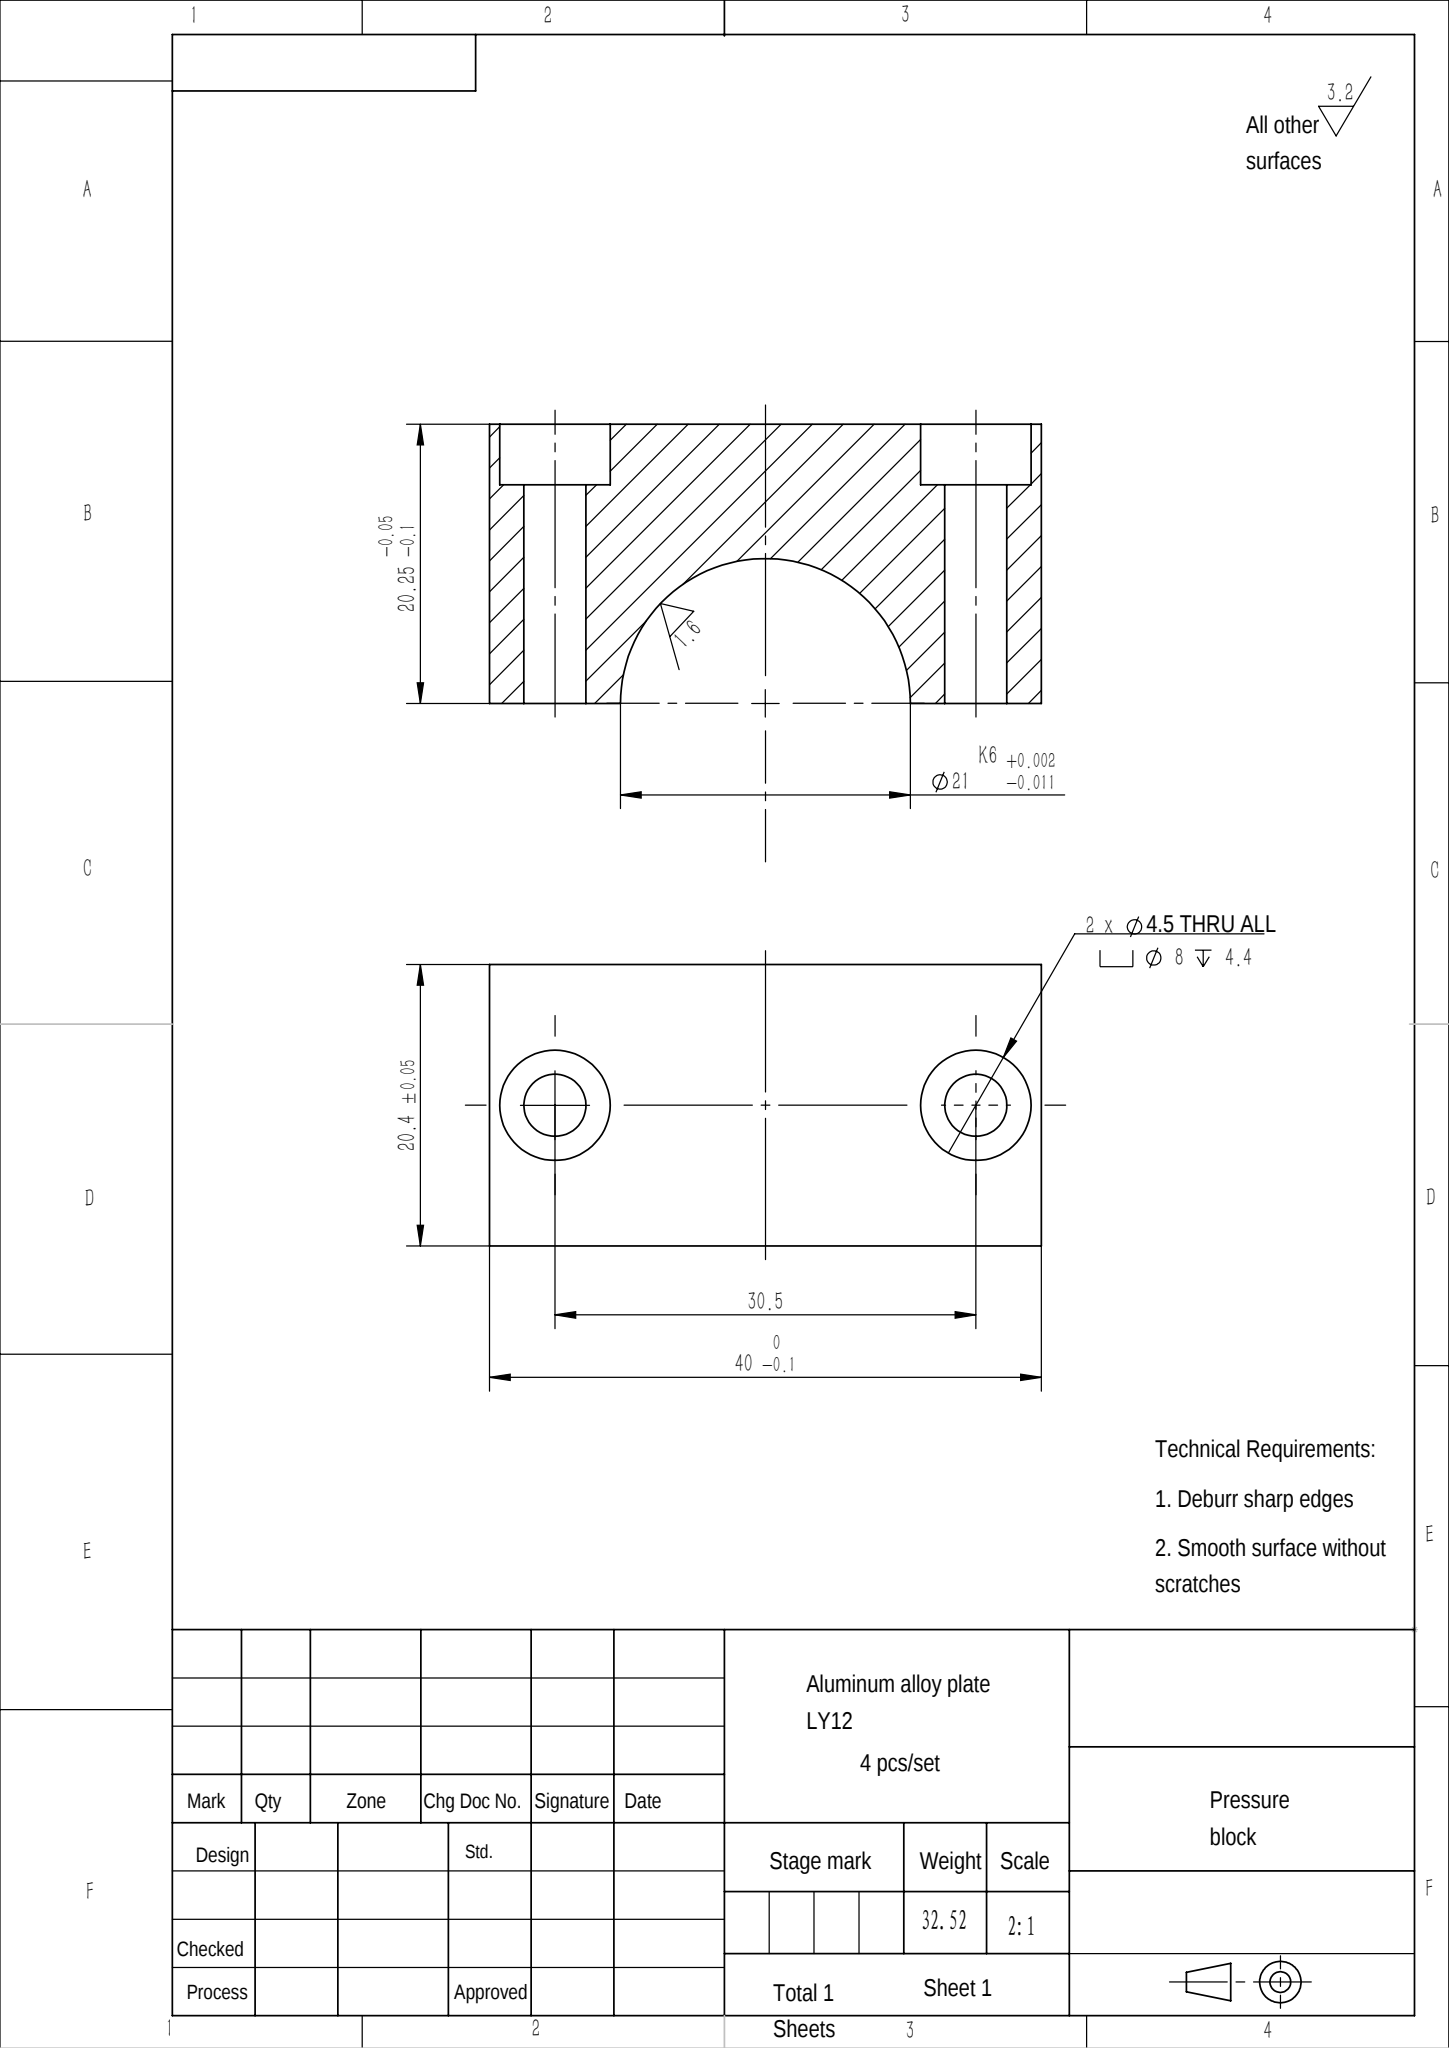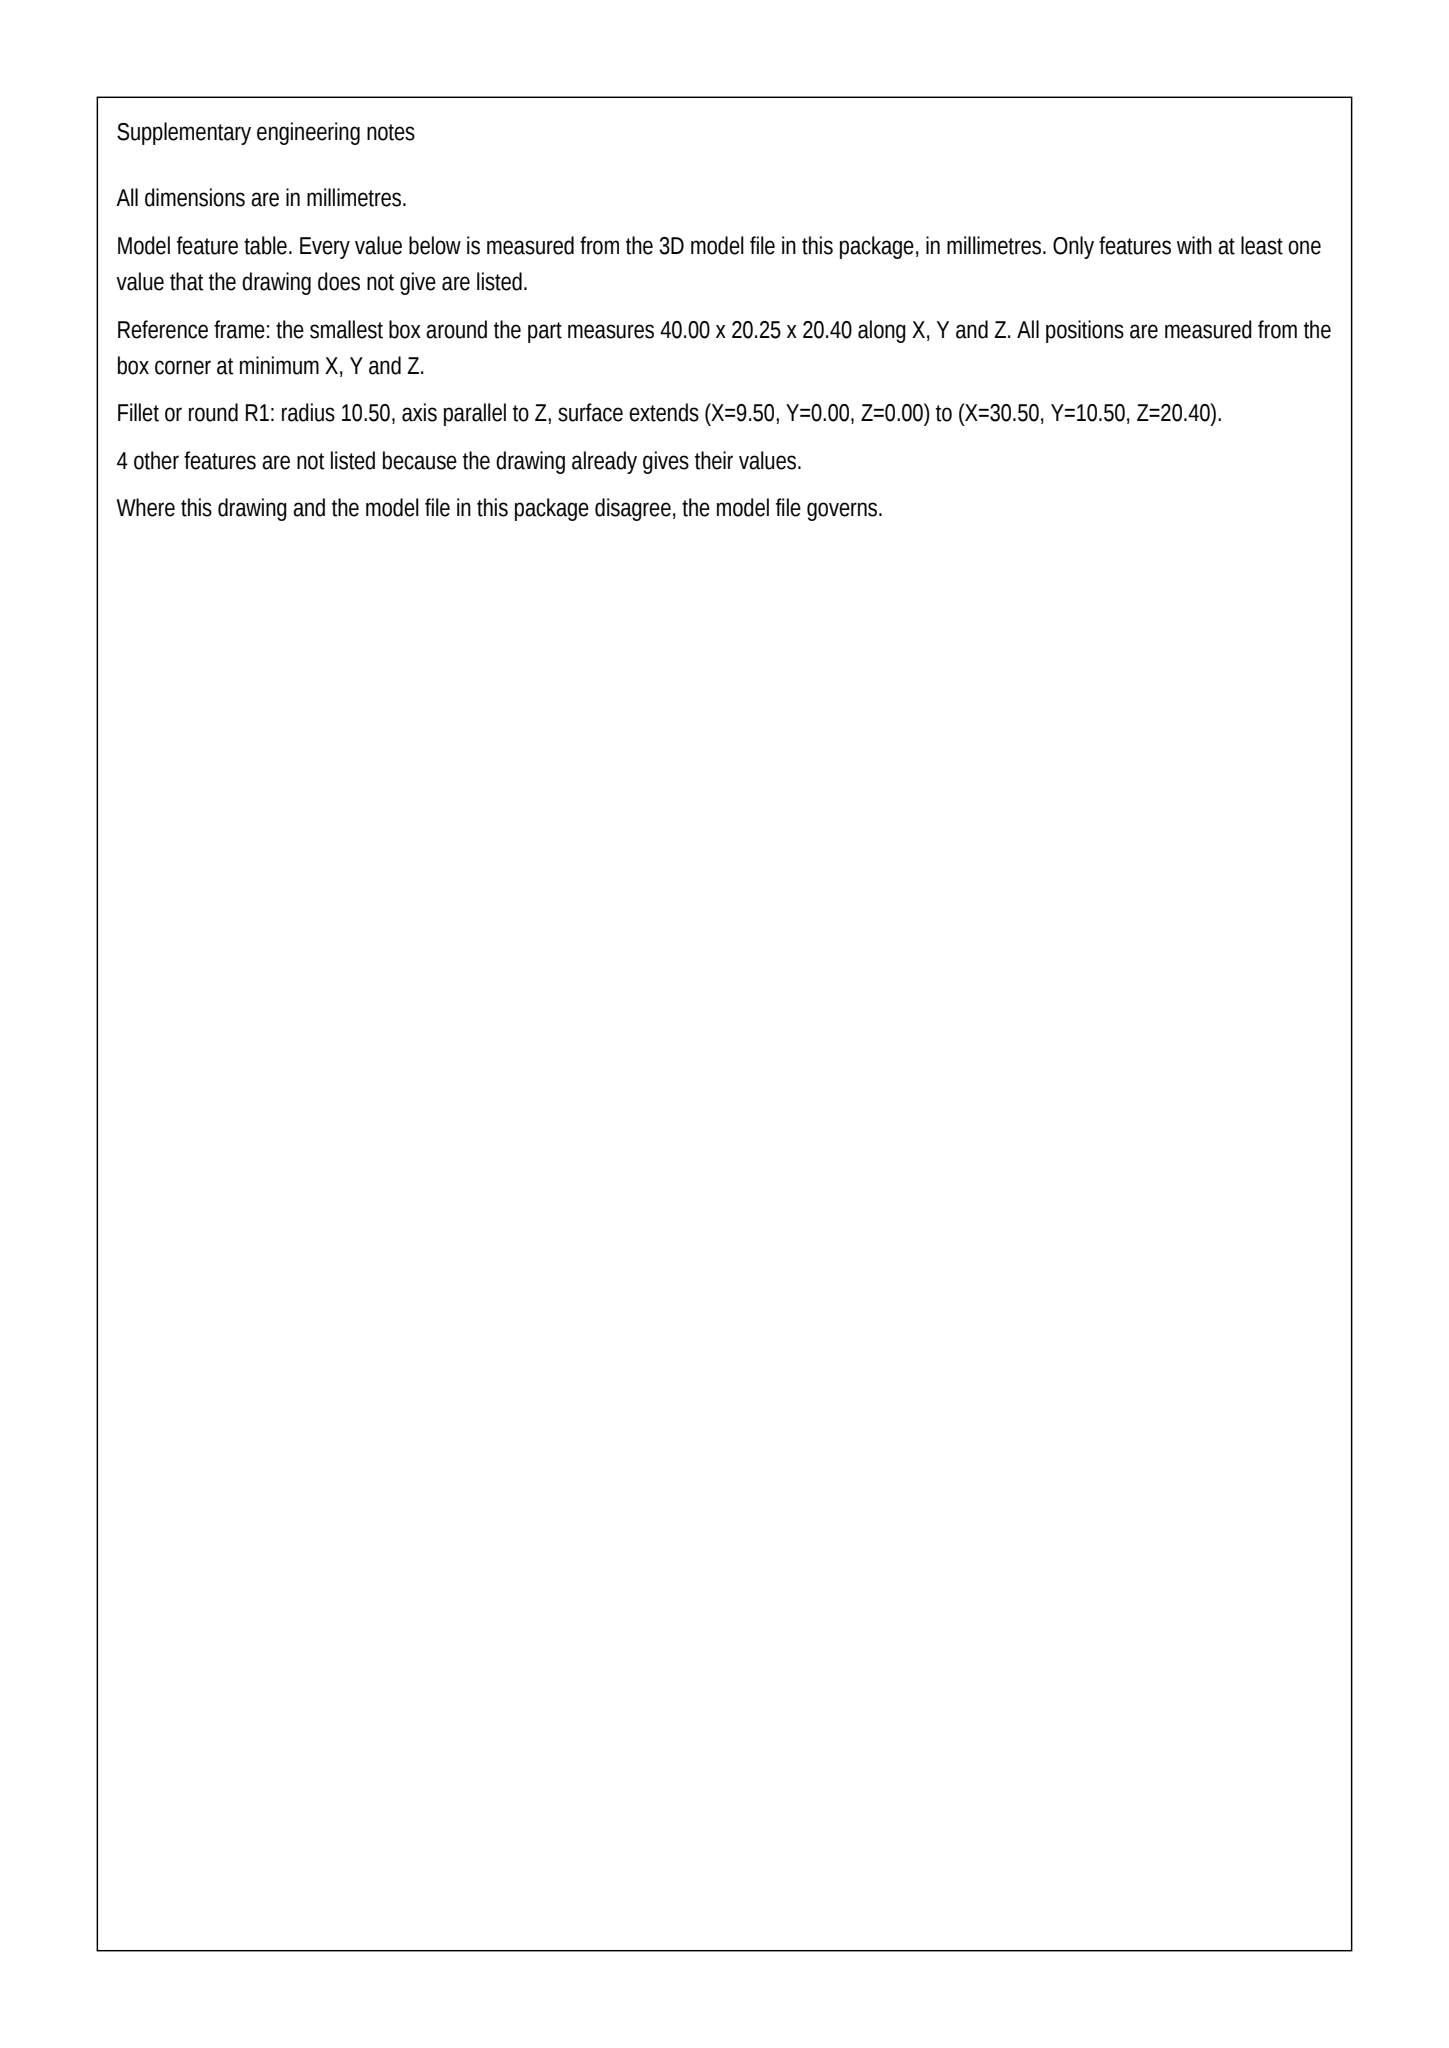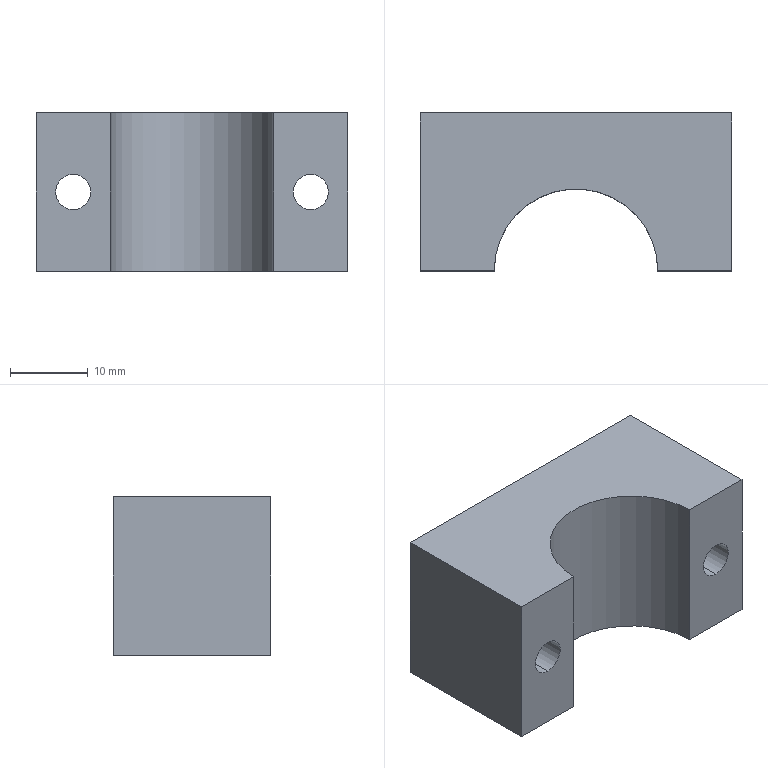Part | SolidWorks | mm | material Aluminum alloy plate LY12 | 1 solid | 18 faces | box 40 x 20.25 x 20.4 mm | volume 12045 mm3 | cylinder 9 | plane 9 | commonest cylinder face diameters 8 x4 4.5 x4 21 x1
build123d program:
from build123d import *

# Parameters (mm, degrees)
SKETCH1_W                                       = 40
SKETCH1_H                                       = 20.25
BOSS_EXTRUDE1_DEPTH                             = 10.2
SKETCH2_R                                       = 10.5
CUT_EXTRUDE1_DEPTH                              = 31.31
M4_HEX_SOCKET_HEAD_CAP_SCREW_CBORE1_D           = 4.5
M4_HEX_SOCKET_HEAD_CAP_SCREW_CBORE1_CBORE_D     = 8
M4_HEX_SOCKET_HEAD_CAP_SCREW_CBORE1_CBORE_DEPTH = 4.4


with BuildPart() as part:
    # Sketch1 → Boss-Extrude1 (new, symmetric)
    with BuildSketch(Plane.XY):
        Rectangle(SKETCH1_W, SKETCH1_H)
    extrude(amount=BOSS_EXTRUDE1_DEPTH, both=True)

    # Sketch2 → Cut-Extrude1 (cut, through all)
    with BuildSketch(Plane.XY.offset(10.2)):
        with Locations((0, -10.125)):
            Circle(SKETCH2_R)
    extrude(amount=-CUT_EXTRUDE1_DEPTH, mode=Mode.SUBTRACT)

    # M4 Hex Socket Head Cap Screw CBORE1 (through all)
    with Locations(Plane(origin=(0, 10.125, 0), x_dir=(1, 0, 0), z_dir=(0, 1, 0))):
        with Locations((-15.25, 0), (15.25, 0)):
            CounterBoreHole(M4_HEX_SOCKET_HEAD_CAP_SCREW_CBORE1_D / 2, M4_HEX_SOCKET_HEAD_CAP_SCREW_CBORE1_CBORE_D / 2, M4_HEX_SOCKET_HEAD_CAP_SCREW_CBORE1_CBORE_DEPTH)


solid = part.part
STEP:
#1=CARTESIAN_POINT('',(-15.25,5.725,-4.));
#2=VERTEX_POINT('',#1);
#3=CARTESIAN_POINT('',(-15.25,5.725,4.));
#4=VERTEX_POINT('',#3);
#5=CARTESIAN_POINT('',(-15.25,5.725,0.));
#6=DIRECTION('',(0.,1.,0.));
#7=DIRECTION('',(0.,0.,1.));
#8=AXIS2_PLACEMENT_3D('',#5,#6,#7);
#9=CIRCLE('',#8,4.);
#10=EDGE_CURVE('',#2,#4,#9,.T.);
#11=ORIENTED_EDGE('',*,*,#10,.F.);
#12=CARTESIAN_POINT('',(-15.25,10.125,-4.));
#13=VERTEX_POINT('',#12);
#14=CARTESIAN_POINT('',(-15.25,10.125,-4.));
#15=DIRECTION('',(0.,1.,0.));
#16=VECTOR('',#15,1000.);
#17=LINE('',#14,#16);
#18=EDGE_CURVE('',#2,#13,#17,.T.);
#19=ORIENTED_EDGE('',*,*,#18,.T.);
#20=CARTESIAN_POINT('',(-15.25,10.125,4.));
#21=VERTEX_POINT('',#20);
#22=CARTESIAN_POINT('',(-15.25,10.125,0.));
#23=DIRECTION('',(0.,1.,0.));
#24=DIRECTION('',(0.,0.,1.));
#25=AXIS2_PLACEMENT_3D('',#22,#23,#24);
#26=CIRCLE('',#25,4.);
#27=EDGE_CURVE('',#13,#21,#26,.T.);
#28=ORIENTED_EDGE('',*,*,#27,.T.);
#29=CARTESIAN_POINT('',(-15.25,10.125,4.));
#30=DIRECTION('',(0.,1.,0.));
#31=VECTOR('',#30,1000.);
#32=LINE('',#29,#31);
#33=EDGE_CURVE('',#4,#21,#32,.T.);
#34=ORIENTED_EDGE('',*,*,#33,.F.);
#35=EDGE_LOOP('',(#11,#19,#28,#34));
#36=FACE_OUTER_BOUND('',#35,.T.);
#37=CARTESIAN_POINT('',(-15.25,10.125,0.));
#38=DIRECTION('',(0.,1.,0.));
#39=DIRECTION('',(0.,0.,1.));
#40=AXIS2_PLACEMENT_3D('',#37,#38,#39);
#41=CYLINDRICAL_SURFACE('',#40,4.);
#42=ADVANCED_FACE('',(#36),#41,.F.);
#43=CARTESIAN_POINT('',(-15.25,-10.125,-2.25));
#44=VERTEX_POINT('',#43);
#45=CARTESIAN_POINT('',(-15.25,-10.125,2.25));
#46=VERTEX_POINT('',#45);
#47=CARTESIAN_POINT('',(-15.25,-10.125,0.));
#48=DIRECTION('',(0.,1.,0.));
#49=DIRECTION('',(0.,0.,1.));
#50=AXIS2_PLACEMENT_3D('',#47,#48,#49);
#51=CIRCLE('',#50,2.25);
#52=EDGE_CURVE('',#44,#46,#51,.T.);
#53=ORIENTED_EDGE('',*,*,#52,.F.);
#54=CARTESIAN_POINT('',(-15.25,5.725,-2.25));
#55=VERTEX_POINT('',#54);
#56=CARTESIAN_POINT('',(-15.25,10.125,-2.25));
#57=DIRECTION('',(0.,1.,0.));
#58=VECTOR('',#57,1000.);
#59=LINE('',#56,#58);
#60=EDGE_CURVE('',#44,#55,#59,.T.);
#61=ORIENTED_EDGE('',*,*,#60,.T.);
#62=CARTESIAN_POINT('',(-15.25,5.725,2.25));
#63=VERTEX_POINT('',#62);
#64=CARTESIAN_POINT('',(-15.25,5.725,0.));
#65=DIRECTION('',(0.,1.,0.));
#66=DIRECTION('',(0.,0.,1.));
#67=AXIS2_PLACEMENT_3D('',#64,#65,#66);
#68=CIRCLE('',#67,2.25);
#69=EDGE_CURVE('',#55,#63,#68,.T.);
#70=ORIENTED_EDGE('',*,*,#69,.T.);
#71=CARTESIAN_POINT('',(-15.25,10.125,2.25));
#72=DIRECTION('',(0.,1.,0.));
#73=VECTOR('',#72,1000.);
#74=LINE('',#71,#73);
#75=EDGE_CURVE('',#46,#63,#74,.T.);
#76=ORIENTED_EDGE('',*,*,#75,.F.);
#77=EDGE_LOOP('',(#53,#61,#70,#76));
#78=FACE_OUTER_BOUND('',#77,.T.);
#79=CARTESIAN_POINT('',(-15.25,10.125,0.));
#80=DIRECTION('',(0.,1.,0.));
#81=DIRECTION('',(0.,0.,1.));
#82=AXIS2_PLACEMENT_3D('',#79,#80,#81);
#83=CYLINDRICAL_SURFACE('',#82,2.25);
#84=ADVANCED_FACE('',(#78),#83,.F.);
#85=CARTESIAN_POINT('',(15.25,5.725,-4.));
#86=VERTEX_POINT('',#85);
#87=CARTESIAN_POINT('',(15.25,5.725,4.));
#88=VERTEX_POINT('',#87);
#89=CARTESIAN_POINT('',(15.25,5.725,0.));
#90=DIRECTION('',(0.,1.,0.));
#91=DIRECTION('',(0.,0.,1.));
#92=AXIS2_PLACEMENT_3D('',#89,#90,#91);
#93=CIRCLE('',#92,4.);
#94=EDGE_CURVE('',#86,#88,#93,.T.);
#95=ORIENTED_EDGE('',*,*,#94,.F.);
#96=CARTESIAN_POINT('',(15.25,10.125,-4.));
#97=VERTEX_POINT('',#96);
#98=CARTESIAN_POINT('',(15.25,10.125,-4.));
#99=DIRECTION('',(0.,1.,0.));
#100=VECTOR('',#99,1000.);
#101=LINE('',#98,#100);
#102=EDGE_CURVE('',#86,#97,#101,.T.);
#103=ORIENTED_EDGE('',*,*,#102,.T.);
#104=CARTESIAN_POINT('',(15.25,10.125,4.));
#105=VERTEX_POINT('',#104);
#106=CARTESIAN_POINT('',(15.25,10.125,0.));
#107=DIRECTION('',(0.,1.,0.));
#108=DIRECTION('',(0.,0.,1.));
#109=AXIS2_PLACEMENT_3D('',#106,#107,#108);
#110=CIRCLE('',#109,4.);
#111=EDGE_CURVE('',#97,#105,#110,.T.);
#112=ORIENTED_EDGE('',*,*,#111,.T.);
#113=CARTESIAN_POINT('',(15.25,10.125,4.));
#114=DIRECTION('',(0.,1.,0.));
#115=VECTOR('',#114,1000.);
#116=LINE('',#113,#115);
#117=EDGE_CURVE('',#88,#105,#116,.T.);
#118=ORIENTED_EDGE('',*,*,#117,.F.);
#119=EDGE_LOOP('',(#95,#103,#112,#118));
#120=FACE_OUTER_BOUND('',#119,.T.);
#121=CARTESIAN_POINT('',(15.25,10.125,0.));
#122=DIRECTION('',(0.,1.,0.));
#123=DIRECTION('',(0.,0.,1.));
#124=AXIS2_PLACEMENT_3D('',#121,#122,#123);
#125=CYLINDRICAL_SURFACE('',#124,4.);
#126=ADVANCED_FACE('',(#120),#125,.F.);
#127=CARTESIAN_POINT('',(15.25,-10.125,-2.25));
#128=VERTEX_POINT('',#127);
#129=CARTESIAN_POINT('',(15.25,-10.125,2.25));
#130=VERTEX_POINT('',#129);
#131=CARTESIAN_POINT('',(15.25,-10.125,0.));
#132=DIRECTION('',(0.,1.,0.));
#133=DIRECTION('',(0.,0.,1.));
#134=AXIS2_PLACEMENT_3D('',#131,#132,#133);
#135=CIRCLE('',#134,2.25);
#136=EDGE_CURVE('',#128,#130,#135,.T.);
#137=ORIENTED_EDGE('',*,*,#136,.F.);
#138=CARTESIAN_POINT('',(15.25,5.725,-2.25));
#139=VERTEX_POINT('',#138);
#140=CARTESIAN_POINT('',(15.25,10.125,-2.25));
#141=DIRECTION('',(0.,1.,0.));
#142=VECTOR('',#141,1000.);
#143=LINE('',#140,#142);
#144=EDGE_CURVE('',#128,#139,#143,.T.);
#145=ORIENTED_EDGE('',*,*,#144,.T.);
#146=CARTESIAN_POINT('',(15.25,5.725,2.25));
#147=VERTEX_POINT('',#146);
#148=CARTESIAN_POINT('',(15.25,5.725,0.));
#149=DIRECTION('',(0.,1.,0.));
#150=DIRECTION('',(0.,0.,1.));
#151=AXIS2_PLACEMENT_3D('',#148,#149,#150);
#152=CIRCLE('',#151,2.25);
#153=EDGE_CURVE('',#139,#147,#152,.T.);
#154=ORIENTED_EDGE('',*,*,#153,.T.);
#155=CARTESIAN_POINT('',(15.25,10.125,2.25));
#156=DIRECTION('',(0.,1.,0.));
#157=VECTOR('',#156,1000.);
#158=LINE('',#155,#157);
#159=EDGE_CURVE('',#130,#147,#158,.T.);
#160=ORIENTED_EDGE('',*,*,#159,.F.);
#161=EDGE_LOOP('',(#137,#145,#154,#160));
#162=FACE_OUTER_BOUND('',#161,.T.);
#163=CARTESIAN_POINT('',(15.25,10.125,0.));
#164=DIRECTION('',(0.,1.,0.));
#165=DIRECTION('',(0.,0.,1.));
#166=AXIS2_PLACEMENT_3D('',#163,#164,#165);
#167=CYLINDRICAL_SURFACE('',#166,2.25);
#168=ADVANCED_FACE('',(#162),#167,.F.);
#169=CARTESIAN_POINT('',(-15.25,-10.125,0.));
#170=DIRECTION('',(0.,1.,0.));
#171=DIRECTION('',(0.,0.,1.));
#172=AXIS2_PLACEMENT_3D('',#169,#170,#171);
#173=CIRCLE('',#172,2.25);
#174=EDGE_CURVE('',#46,#44,#173,.T.);
#175=ORIENTED_EDGE('',*,*,#174,.T.);
#176=ORIENTED_EDGE('',*,*,#52,.T.);
#177=EDGE_LOOP('',(#175,#176));
#178=FACE_BOUND('',#177,.T.);
#179=CARTESIAN_POINT('',(-20.,-10.125,-10.2));
#180=VERTEX_POINT('',#179);
#181=CARTESIAN_POINT('',(-10.5,-10.125,-10.2));
#182=VERTEX_POINT('',#181);
#183=CARTESIAN_POINT('',(-20.,-10.125,-10.2));
#184=DIRECTION('',(1.,0.,0.));
#185=VECTOR('',#184,1000.);
#186=LINE('',#183,#185);
#187=EDGE_CURVE('',#180,#182,#186,.T.);
#188=ORIENTED_EDGE('',*,*,#187,.T.);
#189=CARTESIAN_POINT('',(-10.5,-10.125,10.2));
#190=VERTEX_POINT('',#189);
#191=CARTESIAN_POINT('',(-10.5,-10.125,-10.2));
#192=DIRECTION('',(0.,0.,1.));
#193=VECTOR('',#192,1000.);
#194=LINE('',#191,#193);
#195=EDGE_CURVE('',#182,#190,#194,.T.);
#196=ORIENTED_EDGE('',*,*,#195,.T.);
#197=CARTESIAN_POINT('',(-20.,-10.125,10.2));
#198=VERTEX_POINT('',#197);
#199=CARTESIAN_POINT('',(-20.,-10.125,10.2));
#200=DIRECTION('',(1.,0.,0.));
#201=VECTOR('',#200,1000.);
#202=LINE('',#199,#201);
#203=EDGE_CURVE('',#198,#190,#202,.T.);
#204=ORIENTED_EDGE('',*,*,#203,.F.);
#205=CARTESIAN_POINT('',(-20.,-10.125,10.2));
#206=DIRECTION('',(0.,0.,-1.));
#207=VECTOR('',#206,1000.);
#208=LINE('',#205,#207);
#209=EDGE_CURVE('',#198,#180,#208,.T.);
#210=ORIENTED_EDGE('',*,*,#209,.T.);
#211=EDGE_LOOP('',(#188,#196,#204,#210));
#212=FACE_OUTER_BOUND('',#211,.T.);
#213=CARTESIAN_POINT('',(-20.,-10.125,10.2));
#214=DIRECTION('',(0.,1.,0.));
#215=DIRECTION('',(0.,0.,1.));
#216=AXIS2_PLACEMENT_3D('',#213,#214,#215);
#217=PLANE('',#216);
#218=ADVANCED_FACE('',(#178,#212),#217,.F.);
#219=CARTESIAN_POINT('',(20.,-10.125,-10.2));
#220=VERTEX_POINT('',#219);
#221=CARTESIAN_POINT('',(20.,10.125,-10.2));
#222=VERTEX_POINT('',#221);
#223=CARTESIAN_POINT('',(20.,10.125,-10.2));
#224=DIRECTION('',(0.,1.,0.));
#225=VECTOR('',#224,1000.);
#226=LINE('',#223,#225);
#227=EDGE_CURVE('',#220,#222,#226,.T.);
#228=ORIENTED_EDGE('',*,*,#227,.T.);
#229=CARTESIAN_POINT('',(20.,10.125,10.2));
#230=VERTEX_POINT('',#229);
#231=CARTESIAN_POINT('',(20.,10.125,10.2));
#232=DIRECTION('',(0.,0.,-1.));
#233=VECTOR('',#232,1000.);
#234=LINE('',#231,#233);
#235=EDGE_CURVE('',#230,#222,#234,.T.);
#236=ORIENTED_EDGE('',*,*,#235,.F.);
#237=CARTESIAN_POINT('',(20.,-10.125,10.2));
#238=VERTEX_POINT('',#237);
#239=CARTESIAN_POINT('',(20.,10.125,10.2));
#240=DIRECTION('',(0.,1.,0.));
#241=VECTOR('',#240,1000.);
#242=LINE('',#239,#241);
#243=EDGE_CURVE('',#238,#230,#242,.T.);
#244=ORIENTED_EDGE('',*,*,#243,.F.);
#245=CARTESIAN_POINT('',(20.,-10.125,10.2));
#246=DIRECTION('',(0.,0.,-1.));
#247=VECTOR('',#246,1000.);
#248=LINE('',#245,#247);
#249=EDGE_CURVE('',#238,#220,#248,.T.);
#250=ORIENTED_EDGE('',*,*,#249,.T.);
#251=EDGE_LOOP('',(#228,#236,#244,#250));
#252=FACE_OUTER_BOUND('',#251,.T.);
#253=CARTESIAN_POINT('',(20.,10.125,10.2));
#254=DIRECTION('',(-1.,0.,0.));
#255=DIRECTION('',(0.,0.,1.));
#256=AXIS2_PLACEMENT_3D('',#253,#254,#255);
#257=PLANE('',#256);
#258=ADVANCED_FACE('',(#252),#257,.F.);
#259=CARTESIAN_POINT('',(-15.25,10.125,0.));
#260=DIRECTION('',(0.,1.,0.));
#261=DIRECTION('',(0.,0.,1.));
#262=AXIS2_PLACEMENT_3D('',#259,#260,#261);
#263=CIRCLE('',#262,4.);
#264=EDGE_CURVE('',#21,#13,#263,.T.);
#265=ORIENTED_EDGE('',*,*,#264,.F.);
#266=ORIENTED_EDGE('',*,*,#27,.F.);
#267=EDGE_LOOP('',(#265,#266));
#268=FACE_BOUND('',#267,.T.);
#269=CARTESIAN_POINT('',(15.25,10.125,0.));
#270=DIRECTION('',(0.,1.,0.));
#271=DIRECTION('',(0.,0.,1.));
#272=AXIS2_PLACEMENT_3D('',#269,#270,#271);
#273=CIRCLE('',#272,4.);
#274=EDGE_CURVE('',#105,#97,#273,.T.);
#275=ORIENTED_EDGE('',*,*,#274,.F.);
#276=ORIENTED_EDGE('',*,*,#111,.F.);
#277=EDGE_LOOP('',(#275,#276));
#278=FACE_BOUND('',#277,.T.);
#279=CARTESIAN_POINT('',(-20.,10.125,-10.2));
#280=VERTEX_POINT('',#279);
#281=CARTESIAN_POINT('',(-20.,10.125,-10.2));
#282=DIRECTION('',(-1.,0.,0.));
#283=VECTOR('',#282,1000.);
#284=LINE('',#281,#283);
#285=EDGE_CURVE('',#222,#280,#284,.T.);
#286=ORIENTED_EDGE('',*,*,#285,.T.);
#287=CARTESIAN_POINT('',(-20.,10.125,10.2));
#288=VERTEX_POINT('',#287);
#289=CARTESIAN_POINT('',(-20.,10.125,10.2));
#290=DIRECTION('',(0.,0.,-1.));
#291=VECTOR('',#290,1000.);
#292=LINE('',#289,#291);
#293=EDGE_CURVE('',#288,#280,#292,.T.);
#294=ORIENTED_EDGE('',*,*,#293,.F.);
#295=CARTESIAN_POINT('',(-20.,10.125,10.2));
#296=DIRECTION('',(-1.,0.,0.));
#297=VECTOR('',#296,1000.);
#298=LINE('',#295,#297);
#299=EDGE_CURVE('',#230,#288,#298,.T.);
#300=ORIENTED_EDGE('',*,*,#299,.F.);
#301=ORIENTED_EDGE('',*,*,#235,.T.);
#302=EDGE_LOOP('',(#286,#294,#300,#301));
#303=FACE_OUTER_BOUND('',#302,.T.);
#304=CARTESIAN_POINT('',(-20.,10.125,10.2));
#305=DIRECTION('',(0.,-1.,0.));
#306=DIRECTION('',(0.,0.,-1.));
#307=AXIS2_PLACEMENT_3D('',#304,#305,#306);
#308=PLANE('',#307);
#309=ADVANCED_FACE('',(#268,#278,#303),#308,.F.);
#310=CARTESIAN_POINT('',(-20.,10.125,-10.2));
#311=DIRECTION('',(0.,-1.,0.));
#312=VECTOR('',#311,1000.);
#313=LINE('',#310,#312);
#314=EDGE_CURVE('',#280,#180,#313,.T.);
#315=ORIENTED_EDGE('',*,*,#314,.T.);
#316=ORIENTED_EDGE('',*,*,#209,.F.);
#317=CARTESIAN_POINT('',(-20.,10.125,10.2));
#318=DIRECTION('',(0.,-1.,0.));
#319=VECTOR('',#318,1000.);
#320=LINE('',#317,#319);
#321=EDGE_CURVE('',#288,#198,#320,.T.);
#322=ORIENTED_EDGE('',*,*,#321,.F.);
#323=ORIENTED_EDGE('',*,*,#293,.T.);
#324=EDGE_LOOP('',(#315,#316,#322,#323));
#325=FACE_OUTER_BOUND('',#324,.T.);
#326=CARTESIAN_POINT('',(-20.,10.125,10.2));
#327=DIRECTION('',(1.,0.,0.));
#328=DIRECTION('',(0.,0.,-1.));
#329=AXIS2_PLACEMENT_3D('',#326,#327,#328);
#330=PLANE('',#329);
#331=ADVANCED_FACE('',(#325),#330,.F.);
#332=CARTESIAN_POINT('',(15.25,-10.125,0.));
#333=DIRECTION('',(0.,1.,0.));
#334=DIRECTION('',(0.,0.,1.));
#335=AXIS2_PLACEMENT_3D('',#332,#333,#334);
#336=CIRCLE('',#335,2.25);
#337=EDGE_CURVE('',#130,#128,#336,.T.);
#338=ORIENTED_EDGE('',*,*,#337,.T.);
#339=ORIENTED_EDGE('',*,*,#136,.T.);
#340=EDGE_LOOP('',(#338,#339));
#341=FACE_BOUND('',#340,.T.);
#342=CARTESIAN_POINT('',(10.5,-10.125,10.2));
#343=VERTEX_POINT('',#342);
#344=CARTESIAN_POINT('',(-20.,-10.125,10.2));
#345=DIRECTION('',(1.,0.,0.));
#346=VECTOR('',#345,1000.);
#347=LINE('',#344,#346);
#348=EDGE_CURVE('',#343,#238,#347,.T.);
#349=ORIENTED_EDGE('',*,*,#348,.F.);
#350=CARTESIAN_POINT('',(10.5,-10.125,-10.2));
#351=VERTEX_POINT('',#350);
#352=CARTESIAN_POINT('',(10.5,-10.125,-10.2));
#353=DIRECTION('',(0.,0.,-1.));
#354=VECTOR('',#353,1000.);
#355=LINE('',#352,#354);
#356=EDGE_CURVE('',#343,#351,#355,.T.);
#357=ORIENTED_EDGE('',*,*,#356,.T.);
#358=CARTESIAN_POINT('',(-20.,-10.125,-10.2));
#359=DIRECTION('',(1.,0.,0.));
#360=VECTOR('',#359,1000.);
#361=LINE('',#358,#360);
#362=EDGE_CURVE('',#351,#220,#361,.T.);
#363=ORIENTED_EDGE('',*,*,#362,.T.);
#364=ORIENTED_EDGE('',*,*,#249,.F.);
#365=EDGE_LOOP('',(#349,#357,#363,#364));
#366=FACE_OUTER_BOUND('',#365,.T.);
#367=CARTESIAN_POINT('',(-20.,-10.125,10.2));
#368=DIRECTION('',(0.,1.,0.));
#369=DIRECTION('',(0.,0.,1.));
#370=AXIS2_PLACEMENT_3D('',#367,#368,#369);
#371=PLANE('',#370);
#372=ADVANCED_FACE('',(#341,#366),#371,.F.);
#373=CARTESIAN_POINT('',(0.,-10.125,10.2));
#374=DIRECTION('',(0.,0.,1.));
#375=DIRECTION('',(1.,0.,0.));
#376=AXIS2_PLACEMENT_3D('',#373,#374,#375);
#377=CIRCLE('',#376,10.5);
#378=EDGE_CURVE('',#343,#190,#377,.T.);
#379=ORIENTED_EDGE('',*,*,#378,.F.);
#380=ORIENTED_EDGE('',*,*,#348,.T.);
#381=ORIENTED_EDGE('',*,*,#243,.T.);
#382=ORIENTED_EDGE('',*,*,#299,.T.);
#383=ORIENTED_EDGE('',*,*,#321,.T.);
#384=ORIENTED_EDGE('',*,*,#203,.T.);
#385=EDGE_LOOP('',(#379,#380,#381,#382,#383,#384));
#386=FACE_OUTER_BOUND('',#385,.T.);
#387=CARTESIAN_POINT('',(0.,0.,10.2));
#388=DIRECTION('',(0.,0.,1.));
#389=DIRECTION('',(1.,0.,0.));
#390=AXIS2_PLACEMENT_3D('',#387,#388,#389);
#391=PLANE('',#390);
#392=ADVANCED_FACE('',(#386),#391,.T.);
#393=ORIENTED_EDGE('',*,*,#362,.F.);
#394=CARTESIAN_POINT('',(0.,-10.125,-10.2));
#395=DIRECTION('',(0.,0.,1.));
#396=DIRECTION('',(1.,0.,0.));
#397=AXIS2_PLACEMENT_3D('',#394,#395,#396);
#398=CIRCLE('',#397,10.5);
#399=EDGE_CURVE('',#351,#182,#398,.T.);
#400=ORIENTED_EDGE('',*,*,#399,.T.);
#401=ORIENTED_EDGE('',*,*,#187,.F.);
#402=ORIENTED_EDGE('',*,*,#314,.F.);
#403=ORIENTED_EDGE('',*,*,#285,.F.);
#404=ORIENTED_EDGE('',*,*,#227,.F.);
#405=EDGE_LOOP('',(#393,#400,#401,#402,#403,#404));
#406=FACE_OUTER_BOUND('',#405,.T.);
#407=CARTESIAN_POINT('',(0.,0.,-10.2));
#408=DIRECTION('',(0.,0.,1.));
#409=DIRECTION('',(1.,0.,0.));
#410=AXIS2_PLACEMENT_3D('',#407,#408,#409);
#411=PLANE('',#410);
#412=ADVANCED_FACE('',(#406),#411,.F.);
#413=ORIENTED_EDGE('',*,*,#399,.F.);
#414=ORIENTED_EDGE('',*,*,#356,.F.);
#415=ORIENTED_EDGE('',*,*,#378,.T.);
#416=ORIENTED_EDGE('',*,*,#195,.F.);
#417=EDGE_LOOP('',(#413,#414,#415,#416));
#418=FACE_OUTER_BOUND('',#417,.T.);
#419=CARTESIAN_POINT('',(0.,-10.125,-10.2));
#420=DIRECTION('',(0.,0.,1.));
#421=DIRECTION('',(1.,0.,0.));
#422=AXIS2_PLACEMENT_3D('',#419,#420,#421);
#423=CYLINDRICAL_SURFACE('',#422,10.5);
#424=ADVANCED_FACE('',(#418),#423,.F.);
#425=ORIENTED_EDGE('',*,*,#144,.F.);
#426=ORIENTED_EDGE('',*,*,#337,.F.);
#427=ORIENTED_EDGE('',*,*,#159,.T.);
#428=CARTESIAN_POINT('',(15.25,5.725,0.));
#429=DIRECTION('',(0.,1.,0.));
#430=DIRECTION('',(0.,0.,1.));
#431=AXIS2_PLACEMENT_3D('',#428,#429,#430);
#432=CIRCLE('',#431,2.25);
#433=EDGE_CURVE('',#147,#139,#432,.T.);
#434=ORIENTED_EDGE('',*,*,#433,.T.);
#435=EDGE_LOOP('',(#425,#426,#427,#434));
#436=FACE_OUTER_BOUND('',#435,.T.);
#437=CARTESIAN_POINT('',(15.25,10.125,0.));
#438=DIRECTION('',(0.,1.,0.));
#439=DIRECTION('',(0.,0.,1.));
#440=AXIS2_PLACEMENT_3D('',#437,#438,#439);
#441=CYLINDRICAL_SURFACE('',#440,2.25);
#442=ADVANCED_FACE('',(#436),#441,.F.);
#443=ORIENTED_EDGE('',*,*,#433,.F.);
#444=ORIENTED_EDGE('',*,*,#153,.F.);
#445=EDGE_LOOP('',(#443,#444));
#446=FACE_BOUND('',#445,.T.);
#447=CARTESIAN_POINT('',(15.25,5.725,0.));
#448=DIRECTION('',(0.,1.,0.));
#449=DIRECTION('',(0.,0.,1.));
#450=AXIS2_PLACEMENT_3D('',#447,#448,#449);
#451=CIRCLE('',#450,4.);
#452=EDGE_CURVE('',#88,#86,#451,.T.);
#453=ORIENTED_EDGE('',*,*,#452,.T.);
#454=ORIENTED_EDGE('',*,*,#94,.T.);
#455=EDGE_LOOP('',(#453,#454));
#456=FACE_OUTER_BOUND('',#455,.T.);
#457=CARTESIAN_POINT('',(17.5,5.725,0.));
#458=DIRECTION('',(0.,-1.,0.));
#459=DIRECTION('',(0.,0.,-1.));
#460=AXIS2_PLACEMENT_3D('',#457,#458,#459);
#461=PLANE('',#460);
#462=ADVANCED_FACE('',(#446,#456),#461,.F.);
#463=ORIENTED_EDGE('',*,*,#102,.F.);
#464=ORIENTED_EDGE('',*,*,#452,.F.);
#465=ORIENTED_EDGE('',*,*,#117,.T.);
#466=ORIENTED_EDGE('',*,*,#274,.T.);
#467=EDGE_LOOP('',(#463,#464,#465,#466));
#468=FACE_OUTER_BOUND('',#467,.T.);
#469=CARTESIAN_POINT('',(15.25,10.125,0.));
#470=DIRECTION('',(0.,1.,0.));
#471=DIRECTION('',(0.,0.,1.));
#472=AXIS2_PLACEMENT_3D('',#469,#470,#471);
#473=CYLINDRICAL_SURFACE('',#472,4.);
#474=ADVANCED_FACE('',(#468),#473,.F.);
#475=ORIENTED_EDGE('',*,*,#60,.F.);
#476=ORIENTED_EDGE('',*,*,#174,.F.);
#477=ORIENTED_EDGE('',*,*,#75,.T.);
#478=CARTESIAN_POINT('',(-15.25,5.725,0.));
#479=DIRECTION('',(0.,1.,0.));
#480=DIRECTION('',(0.,0.,1.));
#481=AXIS2_PLACEMENT_3D('',#478,#479,#480);
#482=CIRCLE('',#481,2.25);
#483=EDGE_CURVE('',#63,#55,#482,.T.);
#484=ORIENTED_EDGE('',*,*,#483,.T.);
#485=EDGE_LOOP('',(#475,#476,#477,#484));
#486=FACE_OUTER_BOUND('',#485,.T.);
#487=CARTESIAN_POINT('',(-15.25,10.125,0.));
#488=DIRECTION('',(0.,1.,0.));
#489=DIRECTION('',(0.,0.,1.));
#490=AXIS2_PLACEMENT_3D('',#487,#488,#489);
#491=CYLINDRICAL_SURFACE('',#490,2.25);
#492=ADVANCED_FACE('',(#486),#491,.F.);
#493=ORIENTED_EDGE('',*,*,#483,.F.);
#494=ORIENTED_EDGE('',*,*,#69,.F.);
#495=EDGE_LOOP('',(#493,#494));
#496=FACE_BOUND('',#495,.T.);
#497=CARTESIAN_POINT('',(-15.25,5.725,0.));
#498=DIRECTION('',(0.,1.,0.));
#499=DIRECTION('',(0.,0.,1.));
#500=AXIS2_PLACEMENT_3D('',#497,#498,#499);
#501=CIRCLE('',#500,4.);
#502=EDGE_CURVE('',#4,#2,#501,.T.);
#503=ORIENTED_EDGE('',*,*,#502,.T.);
#504=ORIENTED_EDGE('',*,*,#10,.T.);
#505=EDGE_LOOP('',(#503,#504));
#506=FACE_OUTER_BOUND('',#505,.T.);
#507=CARTESIAN_POINT('',(-13.,5.725,0.));
#508=DIRECTION('',(0.,-1.,0.));
#509=DIRECTION('',(0.,0.,-1.));
#510=AXIS2_PLACEMENT_3D('',#507,#508,#509);
#511=PLANE('',#510);
#512=ADVANCED_FACE('',(#496,#506),#511,.F.);
#513=ORIENTED_EDGE('',*,*,#18,.F.);
#514=ORIENTED_EDGE('',*,*,#502,.F.);
#515=ORIENTED_EDGE('',*,*,#33,.T.);
#516=ORIENTED_EDGE('',*,*,#264,.T.);
#517=EDGE_LOOP('',(#513,#514,#515,#516));
#518=FACE_OUTER_BOUND('',#517,.T.);
#519=CARTESIAN_POINT('',(-15.25,10.125,0.));
#520=DIRECTION('',(0.,1.,0.));
#521=DIRECTION('',(0.,0.,1.));
#522=AXIS2_PLACEMENT_3D('',#519,#520,#521);
#523=CYLINDRICAL_SURFACE('',#522,4.);
#524=ADVANCED_FACE('',(#518),#523,.F.);
#525=CLOSED_SHELL('',(#42,#84,#126,#168,#218,#258,#309,#331,#372,#392,#412,#424,#442,#462,#474,#492,#512,#524));
#526=MANIFOLD_SOLID_BREP('',#525);
#527=CARTESIAN_POINT('',(0.,0.,0.));
#528=DIRECTION('',(0.,0.,1.));
#529=DIRECTION('',(1.,0.,0.));
#530=AXIS2_PLACEMENT_3D('',#527,#528,#529);
#531=(LENGTH_UNIT()NAMED_UNIT(*)SI_UNIT(.MILLI.,.METRE.));
#532=UNCERTAINTY_MEASURE_WITH_UNIT(LENGTH_MEASURE(0.00001),#531,'','');
#533=(NAMED_UNIT(*)PLANE_ANGLE_UNIT()SI_UNIT($,.RADIAN.));
#534=(NAMED_UNIT(*)SI_UNIT($,.STERADIAN.)SOLID_ANGLE_UNIT());
#535=(GEOMETRIC_REPRESENTATION_CONTEXT(3)GLOBAL_UNCERTAINTY_ASSIGNED_CONTEXT((#532))GLOBAL_UNIT_ASSIGNED_CONTEXT((#531,#533,#534))REPRESENTATION_CONTEXT('',''));
#536=ADVANCED_BREP_SHAPE_REPRESENTATION('',(#526,#530),#535);